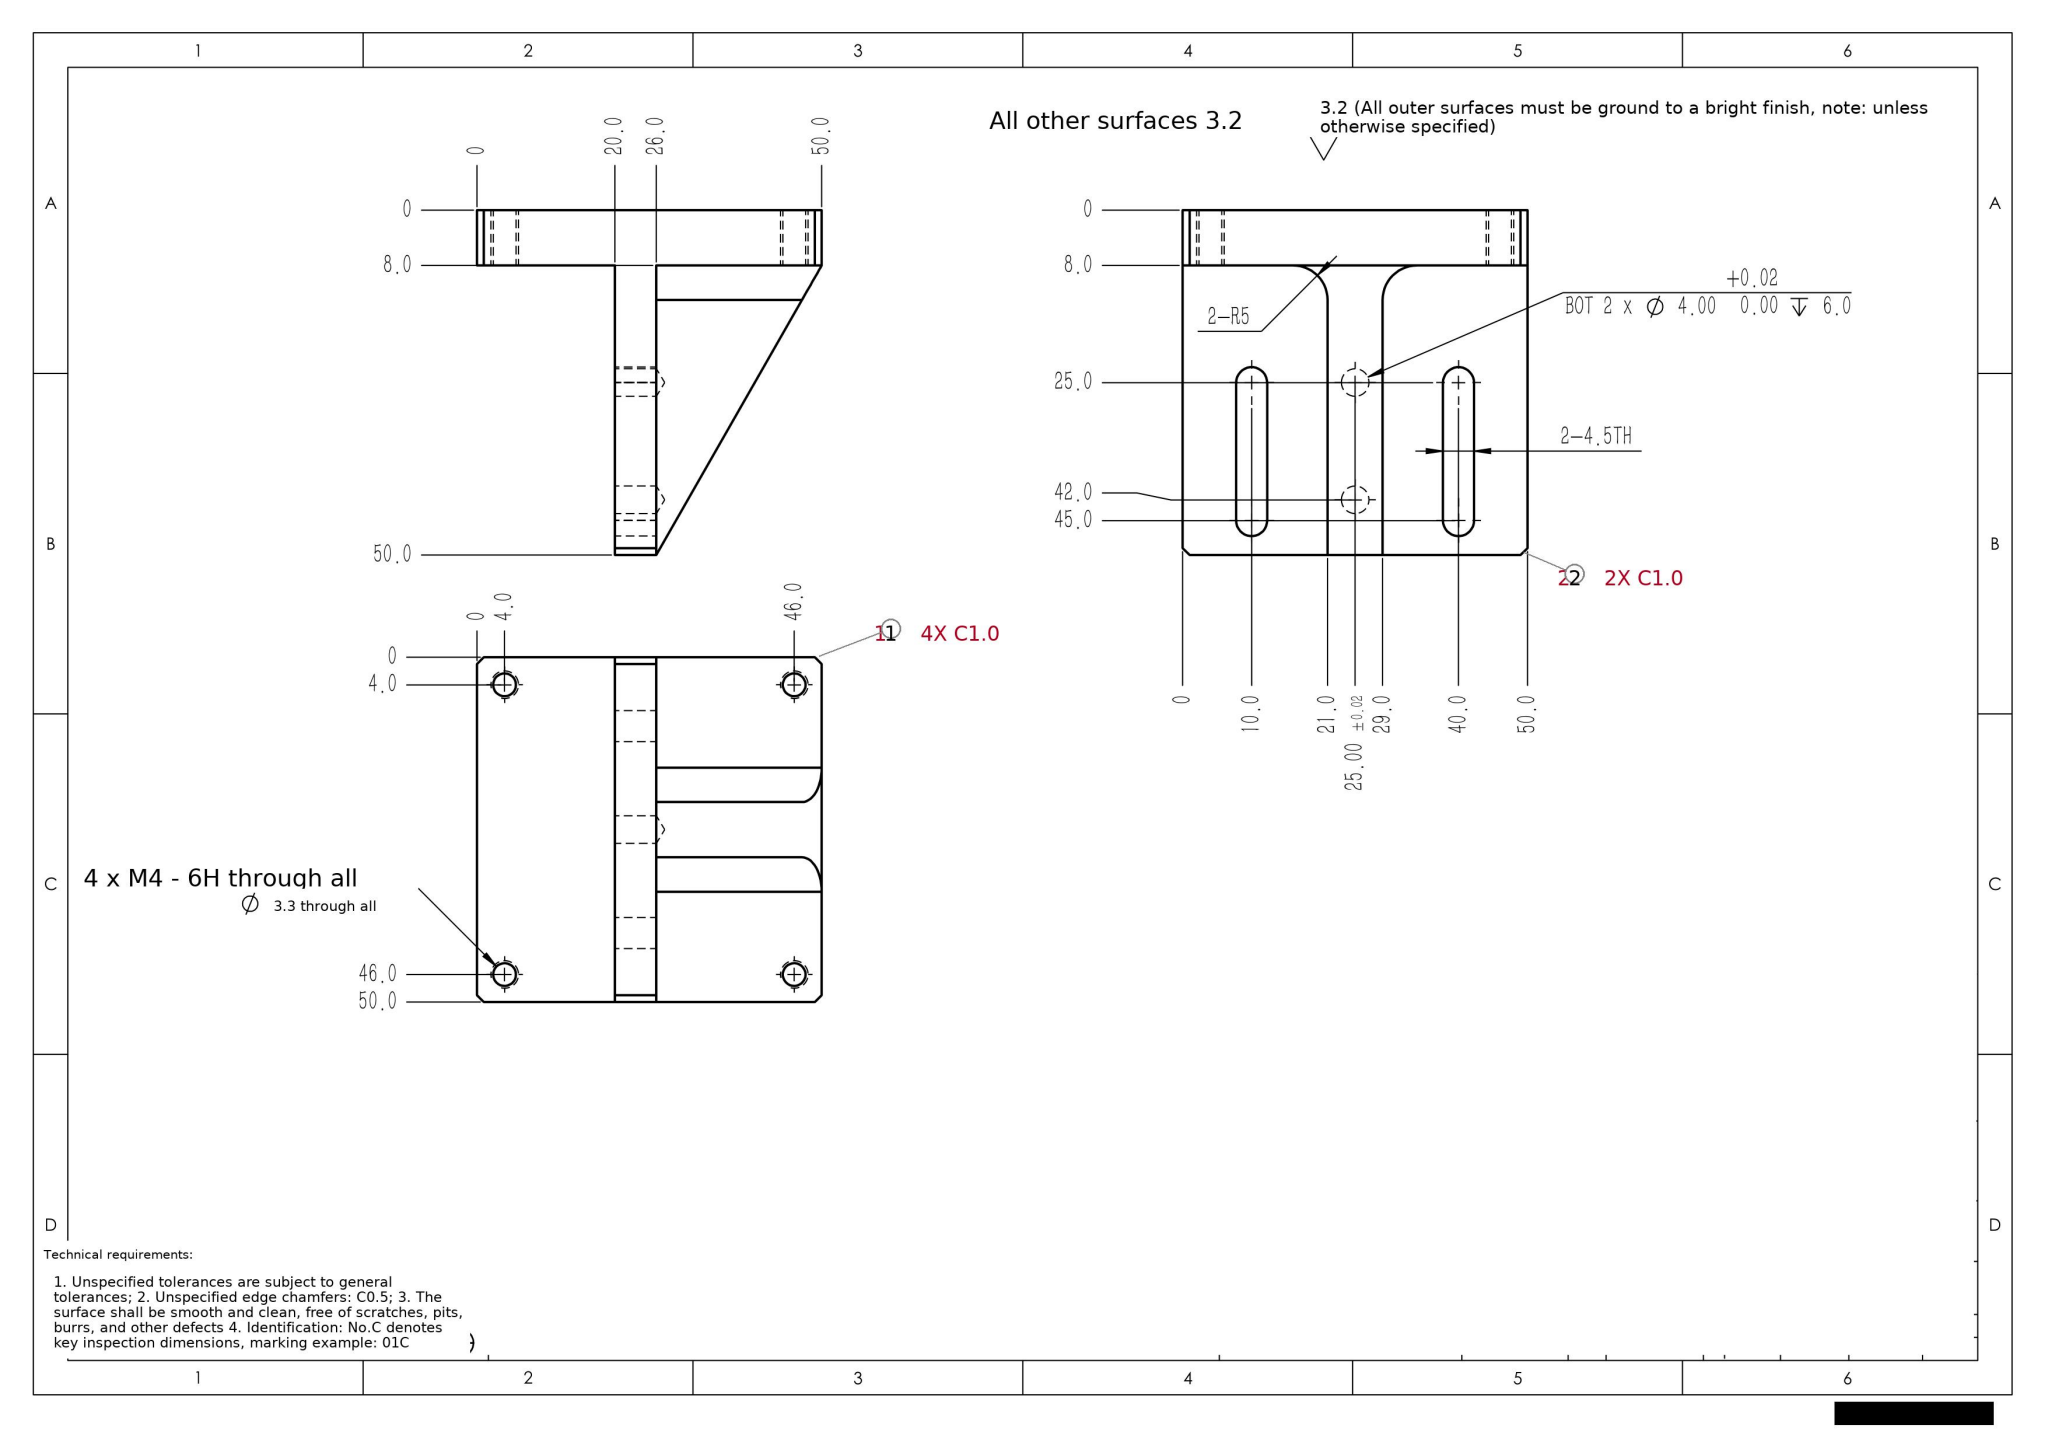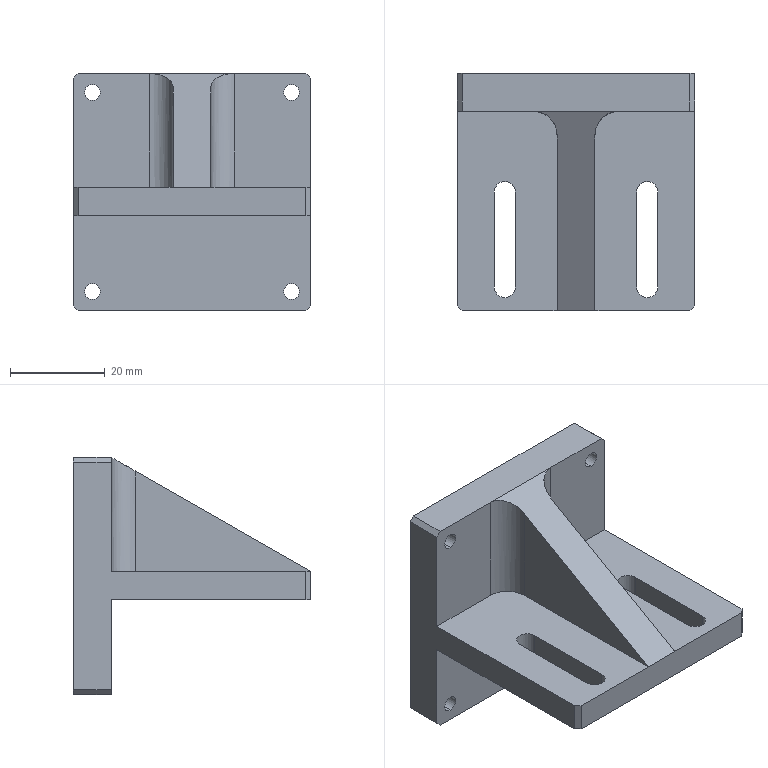Part | SolidWorks | mm | 1 solid | 47 faces | box 50 x 50 x 50 mm | volume 35155 mm3 | plane 25 | cylinder 18 | cone 4 | commonest cylinder face diameters 3.3 x8 4 x4 4.5 x4 10 x2